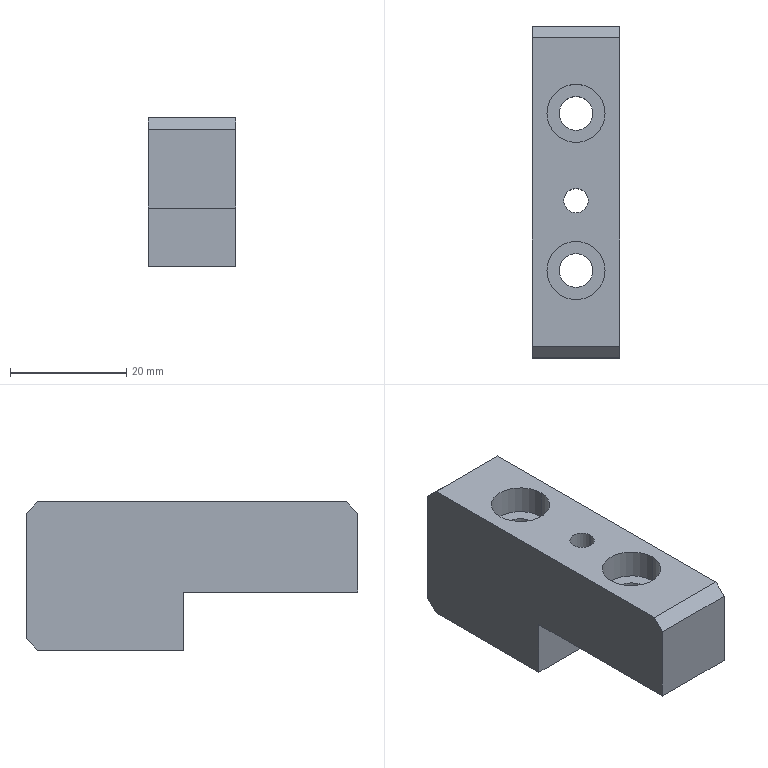Part | SolidWorks | mm | 1 solid | 23 faces | box 15 x 57 x 25.5 mm | volume 15393 mm3 | plane 13 | cylinder 10 | commonest cylinder face diameters 10 x4 5.8 x4 4.2 x2
build123d program:
from build123d import *

# Parameters (mm, degrees)
BOSS_EXTRUDE1_DEPTH                                  = 7.5
COUNTERBORE_FOR_M5_SOCKET_HEAD_CAP_SCREW_D           = 5.8
COUNTERBORE_FOR_M5_SOCKET_HEAD_CAP_SCREW_CBORE_D     = 10
COUNTERBORE_FOR_M5_SOCKET_HEAD_CAP_SCREW_CBORE_DEPTH = 5
M5X0_8_TAPPED_HOLE1_D                                = 4.2
CHAMFER1_SIZE                                        = 2


with BuildPart() as part:
    # Sketch1 → Boss-Extrude1 (new, symmetric)
    with BuildSketch(Plane(origin=(0, 0, 0), x_dir=(0, 0, -1), z_dir=(1, 0, 0))):
        Polygon((0, 0), (0, 57), (25.5, 57), (25.5, 30), (15.5, 30), (15.5, 0), align=None)
    extrude(amount=BOSS_EXTRUDE1_DEPTH, both=True)

    # Counterbore for M5 Socket Head Cap Screw (through all)
    with Locations(Plane.XY):
        with Locations((0, 15), (0, 42)):
            CounterBoreHole(COUNTERBORE_FOR_M5_SOCKET_HEAD_CAP_SCREW_D / 2, COUNTERBORE_FOR_M5_SOCKET_HEAD_CAP_SCREW_CBORE_D / 2, COUNTERBORE_FOR_M5_SOCKET_HEAD_CAP_SCREW_CBORE_DEPTH)

    # M5x0.8 Tapped Hole1 (through all)
    with Locations(Plane.XY):
        with Locations((0, 27)):
            Hole(M5X0_8_TAPPED_HOLE1_D / 2)

    # Chamfer1
    chamfer1_edges = [part.edges().sort_by_distance(p)[0] for p in [
        (0, 0, 0),
        (0, 57, 0),
        (0, 57, -25.5),
    ]]
    chamfer(chamfer1_edges, length=CHAMFER1_SIZE)


solid = part.part
STEP:
#1=CARTESIAN_POINT('',(-2.1,27.,-15.5));
#2=VERTEX_POINT('',#1);
#3=CARTESIAN_POINT('',(2.1,27.,-15.5));
#4=VERTEX_POINT('',#3);
#5=CARTESIAN_POINT('',(0.,27.,-15.5));
#6=DIRECTION('',(0.,-0.,1.));
#7=DIRECTION('',(0.,-1.,0.));
#8=AXIS2_PLACEMENT_3D('',#5,#6,#7);
#9=CIRCLE('',#8,2.1);
#10=EDGE_CURVE('',#2,#4,#9,.T.);
#11=ORIENTED_EDGE('',*,*,#10,.F.);
#12=CARTESIAN_POINT('',(-2.1,27.,0.));
#13=VERTEX_POINT('',#12);
#14=CARTESIAN_POINT('',(-2.1,27.,0.));
#15=DIRECTION('',(0.,0.,1.));
#16=VECTOR('',#15,1000.);
#17=LINE('',#14,#16);
#18=EDGE_CURVE('',#2,#13,#17,.T.);
#19=ORIENTED_EDGE('',*,*,#18,.T.);
#20=CARTESIAN_POINT('',(2.1,27.,0.));
#21=VERTEX_POINT('',#20);
#22=CARTESIAN_POINT('',(0.,27.,0.));
#23=DIRECTION('',(0.,0.,1.));
#24=DIRECTION('',(1.,0.,0.));
#25=AXIS2_PLACEMENT_3D('',#22,#23,#24);
#26=CIRCLE('',#25,2.1);
#27=EDGE_CURVE('',#13,#21,#26,.T.);
#28=ORIENTED_EDGE('',*,*,#27,.T.);
#29=CARTESIAN_POINT('',(2.1,27.,0.));
#30=DIRECTION('',(0.,0.,1.));
#31=VECTOR('',#30,1000.);
#32=LINE('',#29,#31);
#33=EDGE_CURVE('',#4,#21,#32,.T.);
#34=ORIENTED_EDGE('',*,*,#33,.F.);
#35=EDGE_LOOP('',(#11,#19,#28,#34));
#36=FACE_OUTER_BOUND('',#35,.T.);
#37=CARTESIAN_POINT('',(0.,27.,0.));
#38=DIRECTION('',(0.,0.,1.));
#39=DIRECTION('',(1.,0.,0.));
#40=AXIS2_PLACEMENT_3D('',#37,#38,#39);
#41=CYLINDRICAL_SURFACE('',#40,2.1);
#42=ADVANCED_FACE('',(#36),#41,.F.);
#43=CARTESIAN_POINT('',(-5.,15.,-5.));
#44=VERTEX_POINT('',#43);
#45=CARTESIAN_POINT('',(5.,15.,-5.));
#46=VERTEX_POINT('',#45);
#47=CARTESIAN_POINT('',(0.,15.,-5.));
#48=DIRECTION('',(0.,0.,1.));
#49=DIRECTION('',(1.,0.,0.));
#50=AXIS2_PLACEMENT_3D('',#47,#48,#49);
#51=CIRCLE('',#50,5.);
#52=EDGE_CURVE('',#44,#46,#51,.T.);
#53=ORIENTED_EDGE('',*,*,#52,.F.);
#54=CARTESIAN_POINT('',(-5.,15.,0.));
#55=VERTEX_POINT('',#54);
#56=CARTESIAN_POINT('',(-5.,15.,0.));
#57=DIRECTION('',(0.,0.,1.));
#58=VECTOR('',#57,1000.);
#59=LINE('',#56,#58);
#60=EDGE_CURVE('',#44,#55,#59,.T.);
#61=ORIENTED_EDGE('',*,*,#60,.T.);
#62=CARTESIAN_POINT('',(5.,15.,0.));
#63=VERTEX_POINT('',#62);
#64=CARTESIAN_POINT('',(0.,15.,0.));
#65=DIRECTION('',(0.,0.,1.));
#66=DIRECTION('',(1.,0.,0.));
#67=AXIS2_PLACEMENT_3D('',#64,#65,#66);
#68=CIRCLE('',#67,5.);
#69=EDGE_CURVE('',#55,#63,#68,.T.);
#70=ORIENTED_EDGE('',*,*,#69,.T.);
#71=CARTESIAN_POINT('',(5.,15.,0.));
#72=DIRECTION('',(0.,0.,1.));
#73=VECTOR('',#72,1000.);
#74=LINE('',#71,#73);
#75=EDGE_CURVE('',#46,#63,#74,.T.);
#76=ORIENTED_EDGE('',*,*,#75,.F.);
#77=EDGE_LOOP('',(#53,#61,#70,#76));
#78=FACE_OUTER_BOUND('',#77,.T.);
#79=CARTESIAN_POINT('',(0.,15.,0.));
#80=DIRECTION('',(0.,0.,1.));
#81=DIRECTION('',(1.,0.,0.));
#82=AXIS2_PLACEMENT_3D('',#79,#80,#81);
#83=CYLINDRICAL_SURFACE('',#82,5.);
#84=ADVANCED_FACE('',(#78),#83,.F.);
#85=CARTESIAN_POINT('',(-2.9,15.,-15.5));
#86=VERTEX_POINT('',#85);
#87=CARTESIAN_POINT('',(2.9,15.,-15.5));
#88=VERTEX_POINT('',#87);
#89=CARTESIAN_POINT('',(0.,15.,-15.5));
#90=DIRECTION('',(0.,-0.,1.));
#91=DIRECTION('',(0.,-1.,0.));
#92=AXIS2_PLACEMENT_3D('',#89,#90,#91);
#93=CIRCLE('',#92,2.9);
#94=EDGE_CURVE('',#86,#88,#93,.T.);
#95=ORIENTED_EDGE('',*,*,#94,.F.);
#96=CARTESIAN_POINT('',(-2.9,15.,-5.));
#97=VERTEX_POINT('',#96);
#98=CARTESIAN_POINT('',(-2.9,15.,0.));
#99=DIRECTION('',(0.,0.,1.));
#100=VECTOR('',#99,1000.);
#101=LINE('',#98,#100);
#102=EDGE_CURVE('',#86,#97,#101,.T.);
#103=ORIENTED_EDGE('',*,*,#102,.T.);
#104=CARTESIAN_POINT('',(2.9,15.,-5.));
#105=VERTEX_POINT('',#104);
#106=CARTESIAN_POINT('',(0.,15.,-5.));
#107=DIRECTION('',(0.,0.,1.));
#108=DIRECTION('',(1.,0.,0.));
#109=AXIS2_PLACEMENT_3D('',#106,#107,#108);
#110=CIRCLE('',#109,2.9);
#111=EDGE_CURVE('',#97,#105,#110,.T.);
#112=ORIENTED_EDGE('',*,*,#111,.T.);
#113=CARTESIAN_POINT('',(2.9,15.,0.));
#114=DIRECTION('',(0.,0.,1.));
#115=VECTOR('',#114,1000.);
#116=LINE('',#113,#115);
#117=EDGE_CURVE('',#88,#105,#116,.T.);
#118=ORIENTED_EDGE('',*,*,#117,.F.);
#119=EDGE_LOOP('',(#95,#103,#112,#118));
#120=FACE_OUTER_BOUND('',#119,.T.);
#121=CARTESIAN_POINT('',(0.,15.,0.));
#122=DIRECTION('',(0.,0.,1.));
#123=DIRECTION('',(1.,0.,0.));
#124=AXIS2_PLACEMENT_3D('',#121,#122,#123);
#125=CYLINDRICAL_SURFACE('',#124,2.9);
#126=ADVANCED_FACE('',(#120),#125,.F.);
#127=CARTESIAN_POINT('',(-5.,42.,-5.));
#128=VERTEX_POINT('',#127);
#129=CARTESIAN_POINT('',(5.,42.,-5.));
#130=VERTEX_POINT('',#129);
#131=CARTESIAN_POINT('',(0.,42.,-5.));
#132=DIRECTION('',(0.,0.,1.));
#133=DIRECTION('',(1.,0.,0.));
#134=AXIS2_PLACEMENT_3D('',#131,#132,#133);
#135=CIRCLE('',#134,5.);
#136=EDGE_CURVE('',#128,#130,#135,.T.);
#137=ORIENTED_EDGE('',*,*,#136,.F.);
#138=CARTESIAN_POINT('',(-5.,42.,0.));
#139=VERTEX_POINT('',#138);
#140=CARTESIAN_POINT('',(-5.,42.,0.));
#141=DIRECTION('',(0.,0.,1.));
#142=VECTOR('',#141,1000.);
#143=LINE('',#140,#142);
#144=EDGE_CURVE('',#128,#139,#143,.T.);
#145=ORIENTED_EDGE('',*,*,#144,.T.);
#146=CARTESIAN_POINT('',(5.,42.,0.));
#147=VERTEX_POINT('',#146);
#148=CARTESIAN_POINT('',(0.,42.,0.));
#149=DIRECTION('',(0.,0.,1.));
#150=DIRECTION('',(1.,0.,0.));
#151=AXIS2_PLACEMENT_3D('',#148,#149,#150);
#152=CIRCLE('',#151,5.);
#153=EDGE_CURVE('',#139,#147,#152,.T.);
#154=ORIENTED_EDGE('',*,*,#153,.T.);
#155=CARTESIAN_POINT('',(5.,42.,0.));
#156=DIRECTION('',(0.,0.,1.));
#157=VECTOR('',#156,1000.);
#158=LINE('',#155,#157);
#159=EDGE_CURVE('',#130,#147,#158,.T.);
#160=ORIENTED_EDGE('',*,*,#159,.F.);
#161=EDGE_LOOP('',(#137,#145,#154,#160));
#162=FACE_OUTER_BOUND('',#161,.T.);
#163=CARTESIAN_POINT('',(0.,42.,0.));
#164=DIRECTION('',(0.,0.,1.));
#165=DIRECTION('',(1.,0.,0.));
#166=AXIS2_PLACEMENT_3D('',#163,#164,#165);
#167=CYLINDRICAL_SURFACE('',#166,5.);
#168=ADVANCED_FACE('',(#162),#167,.F.);
#169=CARTESIAN_POINT('',(-2.9,42.,-25.5));
#170=VERTEX_POINT('',#169);
#171=CARTESIAN_POINT('',(2.9,42.,-25.5));
#172=VERTEX_POINT('',#171);
#173=CARTESIAN_POINT('',(0.,42.,-25.5));
#174=DIRECTION('',(0.,-0.,1.));
#175=DIRECTION('',(0.,-1.,0.));
#176=AXIS2_PLACEMENT_3D('',#173,#174,#175);
#177=CIRCLE('',#176,2.9);
#178=EDGE_CURVE('',#170,#172,#177,.T.);
#179=ORIENTED_EDGE('',*,*,#178,.F.);
#180=CARTESIAN_POINT('',(-2.9,42.,-5.));
#181=VERTEX_POINT('',#180);
#182=CARTESIAN_POINT('',(-2.9,42.,0.));
#183=DIRECTION('',(0.,0.,1.));
#184=VECTOR('',#183,1000.);
#185=LINE('',#182,#184);
#186=EDGE_CURVE('',#170,#181,#185,.T.);
#187=ORIENTED_EDGE('',*,*,#186,.T.);
#188=CARTESIAN_POINT('',(2.9,42.,-5.));
#189=VERTEX_POINT('',#188);
#190=CARTESIAN_POINT('',(0.,42.,-5.));
#191=DIRECTION('',(0.,0.,1.));
#192=DIRECTION('',(1.,0.,0.));
#193=AXIS2_PLACEMENT_3D('',#190,#191,#192);
#194=CIRCLE('',#193,2.9);
#195=EDGE_CURVE('',#181,#189,#194,.T.);
#196=ORIENTED_EDGE('',*,*,#195,.T.);
#197=CARTESIAN_POINT('',(2.9,42.,0.));
#198=DIRECTION('',(0.,0.,1.));
#199=VECTOR('',#198,1000.);
#200=LINE('',#197,#199);
#201=EDGE_CURVE('',#172,#189,#200,.T.);
#202=ORIENTED_EDGE('',*,*,#201,.F.);
#203=EDGE_LOOP('',(#179,#187,#196,#202));
#204=FACE_OUTER_BOUND('',#203,.T.);
#205=CARTESIAN_POINT('',(0.,42.,0.));
#206=DIRECTION('',(0.,0.,1.));
#207=DIRECTION('',(1.,0.,0.));
#208=AXIS2_PLACEMENT_3D('',#205,#206,#207);
#209=CYLINDRICAL_SURFACE('',#208,2.9);
#210=ADVANCED_FACE('',(#204),#209,.F.);
#211=CARTESIAN_POINT('',(-7.5,55.,0.));
#212=VERTEX_POINT('',#211);
#213=CARTESIAN_POINT('',(-7.5,2.,0.));
#214=VERTEX_POINT('',#213);
#215=CARTESIAN_POINT('',(-7.5,0.,0.));
#216=DIRECTION('',(0.,-1.,0.));
#217=VECTOR('',#216,1000.);
#218=LINE('',#215,#217);
#219=EDGE_CURVE('',#212,#214,#218,.T.);
#220=ORIENTED_EDGE('',*,*,#219,.T.);
#221=CARTESIAN_POINT('',(7.5,2.,0.));
#222=VERTEX_POINT('',#221);
#223=CARTESIAN_POINT('',(7.5,2.,0.));
#224=DIRECTION('',(1.,0.,0.));
#225=VECTOR('',#224,1000.);
#226=LINE('',#223,#225);
#227=EDGE_CURVE('',#214,#222,#226,.T.);
#228=ORIENTED_EDGE('',*,*,#227,.T.);
#229=CARTESIAN_POINT('',(7.5,55.,0.));
#230=VERTEX_POINT('',#229);
#231=CARTESIAN_POINT('',(7.5,0.,0.));
#232=DIRECTION('',(0.,-1.,0.));
#233=VECTOR('',#232,1000.);
#234=LINE('',#231,#233);
#235=EDGE_CURVE('',#230,#222,#234,.T.);
#236=ORIENTED_EDGE('',*,*,#235,.F.);
#237=CARTESIAN_POINT('',(7.5,55.,0.));
#238=DIRECTION('',(-1.,0.,0.));
#239=VECTOR('',#238,1000.);
#240=LINE('',#237,#239);
#241=EDGE_CURVE('',#230,#212,#240,.T.);
#242=ORIENTED_EDGE('',*,*,#241,.T.);
#243=EDGE_LOOP('',(#220,#228,#236,#242));
#244=FACE_OUTER_BOUND('',#243,.T.);
#245=CARTESIAN_POINT('',(0.,42.,0.));
#246=DIRECTION('',(0.,0.,1.));
#247=DIRECTION('',(1.,0.,0.));
#248=AXIS2_PLACEMENT_3D('',#245,#246,#247);
#249=CIRCLE('',#248,5.);
#250=EDGE_CURVE('',#147,#139,#249,.T.);
#251=ORIENTED_EDGE('',*,*,#250,.F.);
#252=ORIENTED_EDGE('',*,*,#153,.F.);
#253=EDGE_LOOP('',(#251,#252));
#254=FACE_BOUND('',#253,.T.);
#255=CARTESIAN_POINT('',(0.,15.,0.));
#256=DIRECTION('',(0.,0.,1.));
#257=DIRECTION('',(1.,0.,0.));
#258=AXIS2_PLACEMENT_3D('',#255,#256,#257);
#259=CIRCLE('',#258,5.);
#260=EDGE_CURVE('',#63,#55,#259,.T.);
#261=ORIENTED_EDGE('',*,*,#260,.F.);
#262=ORIENTED_EDGE('',*,*,#69,.F.);
#263=EDGE_LOOP('',(#261,#262));
#264=FACE_BOUND('',#263,.T.);
#265=CARTESIAN_POINT('',(0.,27.,0.));
#266=DIRECTION('',(0.,0.,1.));
#267=DIRECTION('',(1.,0.,0.));
#268=AXIS2_PLACEMENT_3D('',#265,#266,#267);
#269=CIRCLE('',#268,2.1);
#270=EDGE_CURVE('',#21,#13,#269,.T.);
#271=ORIENTED_EDGE('',*,*,#270,.F.);
#272=ORIENTED_EDGE('',*,*,#27,.F.);
#273=EDGE_LOOP('',(#271,#272));
#274=FACE_BOUND('',#273,.T.);
#275=CARTESIAN_POINT('',(7.5,0.,0.));
#276=DIRECTION('',(0.,0.,-1.));
#277=DIRECTION('',(-1.,0.,0.));
#278=AXIS2_PLACEMENT_3D('',#275,#276,#277);
#279=PLANE('',#278);
#280=ADVANCED_FACE('',(#244,#254,#264,#274),#279,.F.);
#281=CARTESIAN_POINT('',(7.5,-0.,-2.));
#282=VERTEX_POINT('',#281);
#283=CARTESIAN_POINT('',(7.5,-0.,-15.5));
#284=VERTEX_POINT('',#283);
#285=CARTESIAN_POINT('',(7.5,-0.,-15.5));
#286=DIRECTION('',(0.,-0.,-1.));
#287=VECTOR('',#286,1000.);
#288=LINE('',#285,#287);
#289=EDGE_CURVE('',#282,#284,#288,.T.);
#290=ORIENTED_EDGE('',*,*,#289,.F.);
#291=CARTESIAN_POINT('',(-7.5,-0.,-2.));
#292=VERTEX_POINT('',#291);
#293=CARTESIAN_POINT('',(7.5,-0.,-2.));
#294=DIRECTION('',(-1.,0.,0.));
#295=VECTOR('',#294,1000.);
#296=LINE('',#293,#295);
#297=EDGE_CURVE('',#282,#292,#296,.T.);
#298=ORIENTED_EDGE('',*,*,#297,.T.);
#299=CARTESIAN_POINT('',(-7.5,-0.,-15.5));
#300=VERTEX_POINT('',#299);
#301=CARTESIAN_POINT('',(-7.5,-0.,-15.5));
#302=DIRECTION('',(0.,-0.,-1.));
#303=VECTOR('',#302,1000.);
#304=LINE('',#301,#303);
#305=EDGE_CURVE('',#292,#300,#304,.T.);
#306=ORIENTED_EDGE('',*,*,#305,.T.);
#307=CARTESIAN_POINT('',(7.5,-0.,-15.5));
#308=DIRECTION('',(-1.,0.,0.));
#309=VECTOR('',#308,1000.);
#310=LINE('',#307,#309);
#311=EDGE_CURVE('',#284,#300,#310,.T.);
#312=ORIENTED_EDGE('',*,*,#311,.F.);
#313=EDGE_LOOP('',(#290,#298,#306,#312));
#314=FACE_OUTER_BOUND('',#313,.T.);
#315=CARTESIAN_POINT('',(7.5,-0.,-15.5));
#316=DIRECTION('',(0.,1.,-0.));
#317=DIRECTION('',(0.,0.,1.));
#318=AXIS2_PLACEMENT_3D('',#315,#316,#317);
#319=PLANE('',#318);
#320=ADVANCED_FACE('',(#314),#319,.F.);
#321=CARTESIAN_POINT('',(0.,27.,-15.5));
#322=DIRECTION('',(0.,-0.,1.));
#323=DIRECTION('',(0.,-1.,0.));
#324=AXIS2_PLACEMENT_3D('',#321,#322,#323);
#325=CIRCLE('',#324,2.1);
#326=EDGE_CURVE('',#4,#2,#325,.T.);
#327=ORIENTED_EDGE('',*,*,#326,.T.);
#328=ORIENTED_EDGE('',*,*,#10,.T.);
#329=EDGE_LOOP('',(#327,#328));
#330=FACE_BOUND('',#329,.T.);
#331=CARTESIAN_POINT('',(0.,15.,-15.5));
#332=DIRECTION('',(0.,-0.,1.));
#333=DIRECTION('',(0.,-1.,0.));
#334=AXIS2_PLACEMENT_3D('',#331,#332,#333);
#335=CIRCLE('',#334,2.9);
#336=EDGE_CURVE('',#88,#86,#335,.T.);
#337=ORIENTED_EDGE('',*,*,#336,.T.);
#338=ORIENTED_EDGE('',*,*,#94,.T.);
#339=EDGE_LOOP('',(#337,#338));
#340=FACE_BOUND('',#339,.T.);
#341=CARTESIAN_POINT('',(-7.5,30.,-15.5));
#342=VERTEX_POINT('',#341);
#343=CARTESIAN_POINT('',(-7.5,30.,-15.5));
#344=DIRECTION('',(0.,1.,0.));
#345=VECTOR('',#344,1000.);
#346=LINE('',#343,#345);
#347=EDGE_CURVE('',#300,#342,#346,.T.);
#348=ORIENTED_EDGE('',*,*,#347,.T.);
#349=CARTESIAN_POINT('',(7.5,30.,-15.5));
#350=VERTEX_POINT('',#349);
#351=CARTESIAN_POINT('',(7.5,30.,-15.5));
#352=DIRECTION('',(-1.,0.,0.));
#353=VECTOR('',#352,1000.);
#354=LINE('',#351,#353);
#355=EDGE_CURVE('',#350,#342,#354,.T.);
#356=ORIENTED_EDGE('',*,*,#355,.F.);
#357=CARTESIAN_POINT('',(7.5,30.,-15.5));
#358=DIRECTION('',(0.,1.,0.));
#359=VECTOR('',#358,1000.);
#360=LINE('',#357,#359);
#361=EDGE_CURVE('',#284,#350,#360,.T.);
#362=ORIENTED_EDGE('',*,*,#361,.F.);
#363=ORIENTED_EDGE('',*,*,#311,.T.);
#364=EDGE_LOOP('',(#348,#356,#362,#363));
#365=FACE_OUTER_BOUND('',#364,.T.);
#366=CARTESIAN_POINT('',(7.5,30.,-15.5));
#367=DIRECTION('',(0.,-0.,1.));
#368=DIRECTION('',(0.,-1.,-0.));
#369=AXIS2_PLACEMENT_3D('',#366,#367,#368);
#370=PLANE('',#369);
#371=ADVANCED_FACE('',(#330,#340,#365),#370,.F.);
#372=CARTESIAN_POINT('',(-7.5,30.,-25.5));
#373=VERTEX_POINT('',#372);
#374=CARTESIAN_POINT('',(-7.5,30.,-25.5));
#375=DIRECTION('',(0.,0.,-1.));
#376=VECTOR('',#375,1000.);
#377=LINE('',#374,#376);
#378=EDGE_CURVE('',#342,#373,#377,.T.);
#379=ORIENTED_EDGE('',*,*,#378,.T.);
#380=CARTESIAN_POINT('',(7.5,30.,-25.5));
#381=VERTEX_POINT('',#380);
#382=CARTESIAN_POINT('',(7.5,30.,-25.5));
#383=DIRECTION('',(-1.,0.,0.));
#384=VECTOR('',#383,1000.);
#385=LINE('',#382,#384);
#386=EDGE_CURVE('',#381,#373,#385,.T.);
#387=ORIENTED_EDGE('',*,*,#386,.F.);
#388=CARTESIAN_POINT('',(7.5,30.,-25.5));
#389=DIRECTION('',(0.,0.,-1.));
#390=VECTOR('',#389,1000.);
#391=LINE('',#388,#390);
#392=EDGE_CURVE('',#350,#381,#391,.T.);
#393=ORIENTED_EDGE('',*,*,#392,.F.);
#394=ORIENTED_EDGE('',*,*,#355,.T.);
#395=EDGE_LOOP('',(#379,#387,#393,#394));
#396=FACE_OUTER_BOUND('',#395,.T.);
#397=CARTESIAN_POINT('',(7.5,30.,-25.5));
#398=DIRECTION('',(0.,1.,0.));
#399=DIRECTION('',(0.,0.,1.));
#400=AXIS2_PLACEMENT_3D('',#397,#398,#399);
#401=PLANE('',#400);
#402=ADVANCED_FACE('',(#396),#401,.F.);
#403=CARTESIAN_POINT('',(0.,42.,-25.5));
#404=DIRECTION('',(0.,-0.,1.));
#405=DIRECTION('',(0.,-1.,0.));
#406=AXIS2_PLACEMENT_3D('',#403,#404,#405);
#407=CIRCLE('',#406,2.9);
#408=EDGE_CURVE('',#172,#170,#407,.T.);
#409=ORIENTED_EDGE('',*,*,#408,.T.);
#410=ORIENTED_EDGE('',*,*,#178,.T.);
#411=EDGE_LOOP('',(#409,#410));
#412=FACE_BOUND('',#411,.T.);
#413=CARTESIAN_POINT('',(-7.5,55.,-25.5));
#414=VERTEX_POINT('',#413);
#415=CARTESIAN_POINT('',(-7.5,57.,-25.5));
#416=DIRECTION('',(0.,1.,0.));
#417=VECTOR('',#416,1000.);
#418=LINE('',#415,#417);
#419=EDGE_CURVE('',#373,#414,#418,.T.);
#420=ORIENTED_EDGE('',*,*,#419,.T.);
#421=CARTESIAN_POINT('',(7.5,55.,-25.5));
#422=VERTEX_POINT('',#421);
#423=CARTESIAN_POINT('',(7.5,55.,-25.5));
#424=DIRECTION('',(1.,0.,0.));
#425=VECTOR('',#424,1000.);
#426=LINE('',#423,#425);
#427=EDGE_CURVE('',#414,#422,#426,.T.);
#428=ORIENTED_EDGE('',*,*,#427,.T.);
#429=CARTESIAN_POINT('',(7.5,57.,-25.5));
#430=DIRECTION('',(0.,1.,0.));
#431=VECTOR('',#430,1000.);
#432=LINE('',#429,#431);
#433=EDGE_CURVE('',#381,#422,#432,.T.);
#434=ORIENTED_EDGE('',*,*,#433,.F.);
#435=ORIENTED_EDGE('',*,*,#386,.T.);
#436=EDGE_LOOP('',(#420,#428,#434,#435));
#437=FACE_OUTER_BOUND('',#436,.T.);
#438=CARTESIAN_POINT('',(7.5,57.,-25.5));
#439=DIRECTION('',(0.,-0.,1.));
#440=DIRECTION('',(0.,-1.,-0.));
#441=AXIS2_PLACEMENT_3D('',#438,#439,#440);
#442=PLANE('',#441);
#443=ADVANCED_FACE('',(#412,#437),#442,.F.);
#444=CARTESIAN_POINT('',(7.5,57.,-23.5));
#445=VERTEX_POINT('',#444);
#446=CARTESIAN_POINT('',(7.5,57.,-2.));
#447=VERTEX_POINT('',#446);
#448=CARTESIAN_POINT('',(7.5,57.,0.));
#449=DIRECTION('',(0.,0.,1.));
#450=VECTOR('',#449,1000.);
#451=LINE('',#448,#450);
#452=EDGE_CURVE('',#445,#447,#451,.T.);
#453=ORIENTED_EDGE('',*,*,#452,.F.);
#454=CARTESIAN_POINT('',(-7.5,57.,-23.5));
#455=VERTEX_POINT('',#454);
#456=CARTESIAN_POINT('',(7.5,57.,-23.5));
#457=DIRECTION('',(-1.,0.,0.));
#458=VECTOR('',#457,1000.);
#459=LINE('',#456,#458);
#460=EDGE_CURVE('',#445,#455,#459,.T.);
#461=ORIENTED_EDGE('',*,*,#460,.T.);
#462=CARTESIAN_POINT('',(-7.5,57.,-2.));
#463=VERTEX_POINT('',#462);
#464=CARTESIAN_POINT('',(-7.5,57.,0.));
#465=DIRECTION('',(0.,0.,1.));
#466=VECTOR('',#465,1000.);
#467=LINE('',#464,#466);
#468=EDGE_CURVE('',#455,#463,#467,.T.);
#469=ORIENTED_EDGE('',*,*,#468,.T.);
#470=CARTESIAN_POINT('',(7.5,57.,-2.));
#471=DIRECTION('',(1.,0.,0.));
#472=VECTOR('',#471,1000.);
#473=LINE('',#470,#472);
#474=EDGE_CURVE('',#463,#447,#473,.T.);
#475=ORIENTED_EDGE('',*,*,#474,.T.);
#476=EDGE_LOOP('',(#453,#461,#469,#475));
#477=FACE_OUTER_BOUND('',#476,.T.);
#478=CARTESIAN_POINT('',(7.5,57.,0.));
#479=DIRECTION('',(0.,-1.,0.));
#480=DIRECTION('',(0.,0.,-1.));
#481=AXIS2_PLACEMENT_3D('',#478,#479,#480);
#482=PLANE('',#481);
#483=ADVANCED_FACE('',(#477),#482,.F.);
#484=ORIENTED_EDGE('',*,*,#235,.T.);
#485=CARTESIAN_POINT('',(7.5,-0.,-2.));
#486=DIRECTION('',(0.,-0.7071,-0.7071));
#487=VECTOR('',#486,1000.);
#488=LINE('',#485,#487);
#489=EDGE_CURVE('',#222,#282,#488,.T.);
#490=ORIENTED_EDGE('',*,*,#489,.T.);
#491=ORIENTED_EDGE('',*,*,#289,.T.);
#492=ORIENTED_EDGE('',*,*,#361,.T.);
#493=ORIENTED_EDGE('',*,*,#392,.T.);
#494=ORIENTED_EDGE('',*,*,#433,.T.);
#495=CARTESIAN_POINT('',(7.5,57.,-23.5));
#496=DIRECTION('',(0.,0.7071,0.7071));
#497=VECTOR('',#496,1000.);
#498=LINE('',#495,#497);
#499=EDGE_CURVE('',#422,#445,#498,.T.);
#500=ORIENTED_EDGE('',*,*,#499,.T.);
#501=ORIENTED_EDGE('',*,*,#452,.T.);
#502=CARTESIAN_POINT('',(7.5,55.,0.));
#503=DIRECTION('',(0.,-0.7071,0.7071));
#504=VECTOR('',#503,1000.);
#505=LINE('',#502,#504);
#506=EDGE_CURVE('',#447,#230,#505,.T.);
#507=ORIENTED_EDGE('',*,*,#506,.T.);
#508=EDGE_LOOP('',(#484,#490,#491,#492,#493,#494,#500,#501,#507));
#509=FACE_OUTER_BOUND('',#508,.T.);
#510=CARTESIAN_POINT('',(7.5,0.,0.));
#511=DIRECTION('',(-1.,0.,0.));
#512=DIRECTION('',(0.,0.,1.));
#513=AXIS2_PLACEMENT_3D('',#510,#511,#512);
#514=PLANE('',#513);
#515=ADVANCED_FACE('',(#509),#514,.F.);
#516=ORIENTED_EDGE('',*,*,#305,.F.);
#517=CARTESIAN_POINT('',(-7.5,1.,-1.));
#518=DIRECTION('',(0.,0.7071,0.7071));
#519=VECTOR('',#518,1000.);
#520=LINE('',#517,#519);
#521=EDGE_CURVE('',#292,#214,#520,.T.);
#522=ORIENTED_EDGE('',*,*,#521,.T.);
#523=ORIENTED_EDGE('',*,*,#219,.F.);
#524=CARTESIAN_POINT('',(-7.5,27.5,27.5));
#525=DIRECTION('',(0.,0.7071,-0.7071));
#526=VECTOR('',#525,1000.);
#527=LINE('',#524,#526);
#528=EDGE_CURVE('',#212,#463,#527,.T.);
#529=ORIENTED_EDGE('',*,*,#528,.T.);
#530=ORIENTED_EDGE('',*,*,#468,.F.);
#531=CARTESIAN_POINT('',(-7.5,40.25,-40.25));
#532=DIRECTION('',(0.,-0.7071,-0.7071));
#533=VECTOR('',#532,1000.);
#534=LINE('',#531,#533);
#535=EDGE_CURVE('',#455,#414,#534,.T.);
#536=ORIENTED_EDGE('',*,*,#535,.T.);
#537=ORIENTED_EDGE('',*,*,#419,.F.);
#538=ORIENTED_EDGE('',*,*,#378,.F.);
#539=ORIENTED_EDGE('',*,*,#347,.F.);
#540=EDGE_LOOP('',(#516,#522,#523,#529,#530,#536,#537,#538,#539));
#541=FACE_OUTER_BOUND('',#540,.T.);
#542=CARTESIAN_POINT('',(-7.5,0.,0.));
#543=DIRECTION('',(-1.,0.,0.));
#544=DIRECTION('',(0.,0.,1.));
#545=AXIS2_PLACEMENT_3D('',#542,#543,#544);
#546=PLANE('',#545);
#547=ADVANCED_FACE('',(#541),#546,.T.);
#548=ORIENTED_EDGE('',*,*,#186,.F.);
#549=ORIENTED_EDGE('',*,*,#408,.F.);
#550=ORIENTED_EDGE('',*,*,#201,.T.);
#551=CARTESIAN_POINT('',(0.,42.,-5.));
#552=DIRECTION('',(0.,0.,1.));
#553=DIRECTION('',(1.,0.,0.));
#554=AXIS2_PLACEMENT_3D('',#551,#552,#553);
#555=CIRCLE('',#554,2.9);
#556=EDGE_CURVE('',#189,#181,#555,.T.);
#557=ORIENTED_EDGE('',*,*,#556,.T.);
#558=EDGE_LOOP('',(#548,#549,#550,#557));
#559=FACE_OUTER_BOUND('',#558,.T.);
#560=CARTESIAN_POINT('',(0.,42.,0.));
#561=DIRECTION('',(0.,0.,1.));
#562=DIRECTION('',(1.,0.,0.));
#563=AXIS2_PLACEMENT_3D('',#560,#561,#562);
#564=CYLINDRICAL_SURFACE('',#563,2.9);
#565=ADVANCED_FACE('',(#559),#564,.F.);
#566=ORIENTED_EDGE('',*,*,#556,.F.);
#567=ORIENTED_EDGE('',*,*,#195,.F.);
#568=EDGE_LOOP('',(#566,#567));
#569=FACE_BOUND('',#568,.T.);
#570=CARTESIAN_POINT('',(0.,42.,-5.));
#571=DIRECTION('',(0.,0.,1.));
#572=DIRECTION('',(1.,0.,0.));
#573=AXIS2_PLACEMENT_3D('',#570,#571,#572);
#574=CIRCLE('',#573,5.);
#575=EDGE_CURVE('',#130,#128,#574,.T.);
#576=ORIENTED_EDGE('',*,*,#575,.T.);
#577=ORIENTED_EDGE('',*,*,#136,.T.);
#578=EDGE_LOOP('',(#576,#577));
#579=FACE_OUTER_BOUND('',#578,.T.);
#580=CARTESIAN_POINT('',(2.9,42.,-5.));
#581=DIRECTION('',(0.,0.,-1.));
#582=DIRECTION('',(-1.,0.,0.));
#583=AXIS2_PLACEMENT_3D('',#580,#581,#582);
#584=PLANE('',#583);
#585=ADVANCED_FACE('',(#569,#579),#584,.F.);
#586=ORIENTED_EDGE('',*,*,#144,.F.);
#587=ORIENTED_EDGE('',*,*,#575,.F.);
#588=ORIENTED_EDGE('',*,*,#159,.T.);
#589=ORIENTED_EDGE('',*,*,#250,.T.);
#590=EDGE_LOOP('',(#586,#587,#588,#589));
#591=FACE_OUTER_BOUND('',#590,.T.);
#592=CARTESIAN_POINT('',(0.,42.,0.));
#593=DIRECTION('',(0.,0.,1.));
#594=DIRECTION('',(1.,0.,0.));
#595=AXIS2_PLACEMENT_3D('',#592,#593,#594);
#596=CYLINDRICAL_SURFACE('',#595,5.);
#597=ADVANCED_FACE('',(#591),#596,.F.);
#598=ORIENTED_EDGE('',*,*,#102,.F.);
#599=ORIENTED_EDGE('',*,*,#336,.F.);
#600=ORIENTED_EDGE('',*,*,#117,.T.);
#601=CARTESIAN_POINT('',(0.,15.,-5.));
#602=DIRECTION('',(0.,0.,1.));
#603=DIRECTION('',(1.,0.,0.));
#604=AXIS2_PLACEMENT_3D('',#601,#602,#603);
#605=CIRCLE('',#604,2.9);
#606=EDGE_CURVE('',#105,#97,#605,.T.);
#607=ORIENTED_EDGE('',*,*,#606,.T.);
#608=EDGE_LOOP('',(#598,#599,#600,#607));
#609=FACE_OUTER_BOUND('',#608,.T.);
#610=CARTESIAN_POINT('',(0.,15.,0.));
#611=DIRECTION('',(0.,0.,1.));
#612=DIRECTION('',(1.,0.,0.));
#613=AXIS2_PLACEMENT_3D('',#610,#611,#612);
#614=CYLINDRICAL_SURFACE('',#613,2.9);
#615=ADVANCED_FACE('',(#609),#614,.F.);
#616=ORIENTED_EDGE('',*,*,#606,.F.);
#617=ORIENTED_EDGE('',*,*,#111,.F.);
#618=EDGE_LOOP('',(#616,#617));
#619=FACE_BOUND('',#618,.T.);
#620=CARTESIAN_POINT('',(0.,15.,-5.));
#621=DIRECTION('',(0.,0.,1.));
#622=DIRECTION('',(1.,0.,0.));
#623=AXIS2_PLACEMENT_3D('',#620,#621,#622);
#624=CIRCLE('',#623,5.);
#625=EDGE_CURVE('',#46,#44,#624,.T.);
#626=ORIENTED_EDGE('',*,*,#625,.T.);
#627=ORIENTED_EDGE('',*,*,#52,.T.);
#628=EDGE_LOOP('',(#626,#627));
#629=FACE_OUTER_BOUND('',#628,.T.);
#630=CARTESIAN_POINT('',(2.9,15.,-5.));
#631=DIRECTION('',(0.,0.,-1.));
#632=DIRECTION('',(-1.,0.,0.));
#633=AXIS2_PLACEMENT_3D('',#630,#631,#632);
#634=PLANE('',#633);
#635=ADVANCED_FACE('',(#619,#629),#634,.F.);
#636=ORIENTED_EDGE('',*,*,#60,.F.);
#637=ORIENTED_EDGE('',*,*,#625,.F.);
#638=ORIENTED_EDGE('',*,*,#75,.T.);
#639=ORIENTED_EDGE('',*,*,#260,.T.);
#640=EDGE_LOOP('',(#636,#637,#638,#639));
#641=FACE_OUTER_BOUND('',#640,.T.);
#642=CARTESIAN_POINT('',(0.,15.,0.));
#643=DIRECTION('',(0.,0.,1.));
#644=DIRECTION('',(1.,0.,0.));
#645=AXIS2_PLACEMENT_3D('',#642,#643,#644);
#646=CYLINDRICAL_SURFACE('',#645,5.);
#647=ADVANCED_FACE('',(#641),#646,.F.);
#648=ORIENTED_EDGE('',*,*,#18,.F.);
#649=ORIENTED_EDGE('',*,*,#326,.F.);
#650=ORIENTED_EDGE('',*,*,#33,.T.);
#651=ORIENTED_EDGE('',*,*,#270,.T.);
#652=EDGE_LOOP('',(#648,#649,#650,#651));
#653=FACE_OUTER_BOUND('',#652,.T.);
#654=CARTESIAN_POINT('',(0.,27.,0.));
#655=DIRECTION('',(0.,0.,1.));
#656=DIRECTION('',(1.,0.,0.));
#657=AXIS2_PLACEMENT_3D('',#654,#655,#656);
#658=CYLINDRICAL_SURFACE('',#657,2.1);
#659=ADVANCED_FACE('',(#653),#658,.F.);
#660=ORIENTED_EDGE('',*,*,#489,.F.);
#661=ORIENTED_EDGE('',*,*,#227,.F.);
#662=ORIENTED_EDGE('',*,*,#521,.F.);
#663=ORIENTED_EDGE('',*,*,#297,.F.);
#664=EDGE_LOOP('',(#660,#661,#662,#663));
#665=FACE_OUTER_BOUND('',#664,.T.);
#666=CARTESIAN_POINT('',(7.5,-0.,-2.));
#667=DIRECTION('',(0.,0.7071,-0.7071));
#668=DIRECTION('',(-1.,0.,0.));
#669=AXIS2_PLACEMENT_3D('',#666,#667,#668);
#670=PLANE('',#669);
#671=ADVANCED_FACE('',(#665),#670,.F.);
#672=ORIENTED_EDGE('',*,*,#499,.F.);
#673=ORIENTED_EDGE('',*,*,#427,.F.);
#674=ORIENTED_EDGE('',*,*,#535,.F.);
#675=ORIENTED_EDGE('',*,*,#460,.F.);
#676=EDGE_LOOP('',(#672,#673,#674,#675));
#677=FACE_OUTER_BOUND('',#676,.T.);
#678=CARTESIAN_POINT('',(7.5,57.,-23.5));
#679=DIRECTION('',(0.,-0.7071,0.7071));
#680=DIRECTION('',(-1.,0.,0.));
#681=AXIS2_PLACEMENT_3D('',#678,#679,#680);
#682=PLANE('',#681);
#683=ADVANCED_FACE('',(#677),#682,.F.);
#684=ORIENTED_EDGE('',*,*,#506,.F.);
#685=ORIENTED_EDGE('',*,*,#474,.F.);
#686=ORIENTED_EDGE('',*,*,#528,.F.);
#687=ORIENTED_EDGE('',*,*,#241,.F.);
#688=EDGE_LOOP('',(#684,#685,#686,#687));
#689=FACE_OUTER_BOUND('',#688,.T.);
#690=CARTESIAN_POINT('',(7.5,55.,0.));
#691=DIRECTION('',(0.,-0.7071,-0.7071));
#692=DIRECTION('',(-1.,0.,0.));
#693=AXIS2_PLACEMENT_3D('',#690,#691,#692);
#694=PLANE('',#693);
#695=ADVANCED_FACE('',(#689),#694,.F.);
#696=CLOSED_SHELL('',(#42,#84,#126,#168,#210,#280,#320,#371,#402,#443,#483,#515,#547,#565,#585,#597,#615,#635,#647,#659,#671,#683,#695));
#697=MANIFOLD_SOLID_BREP('',#696);
#698=CARTESIAN_POINT('',(0.,0.,0.));
#699=DIRECTION('',(0.,0.,1.));
#700=DIRECTION('',(1.,0.,0.));
#701=AXIS2_PLACEMENT_3D('',#698,#699,#700);
#702=(LENGTH_UNIT()NAMED_UNIT(*)SI_UNIT(.MILLI.,.METRE.));
#703=UNCERTAINTY_MEASURE_WITH_UNIT(LENGTH_MEASURE(0.00001),#702,'','');
#704=(NAMED_UNIT(*)PLANE_ANGLE_UNIT()SI_UNIT($,.RADIAN.));
#705=(NAMED_UNIT(*)SI_UNIT($,.STERADIAN.)SOLID_ANGLE_UNIT());
#706=(GEOMETRIC_REPRESENTATION_CONTEXT(3)GLOBAL_UNCERTAINTY_ASSIGNED_CONTEXT((#703))GLOBAL_UNIT_ASSIGNED_CONTEXT((#702,#704,#705))REPRESENTATION_CONTEXT('',''));
#707=ADVANCED_BREP_SHAPE_REPRESENTATION('',(#697,#701),#706);